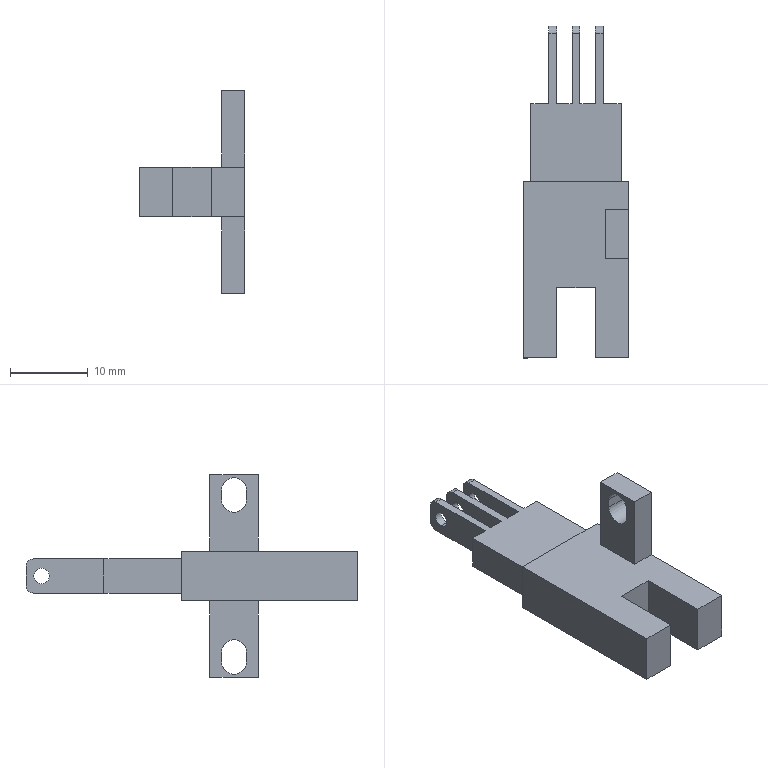Component | SolidWorks | U-shapedSensor8.28-1 | 1 solid | 55 faces | box 13.6 x 42.6 x 26 mm | volume 2610 mm3 | plane 39 | cylinder 16 | commonest cylinder face diameters 2 x12 3.2 x4
build123d program:
from build123d import *

# Parameters (mm, degrees)
SKETCH1_W              = 13.6
SKETCH1_H              = 22.6
BOSS_EXTRUDE1_DEPTH    = 6.4
SKETCH2_W              = 4.9
SKETCH2_H              = 9
CUT_EXTRUDE1_DEPTH     = 28.142
SKETCH3_W              = 13
SKETCH3_H              = 6.2
BOSS_EXTRUDE2_DEPTH    = 3
CUT_EXTRUDE2_DEPTH     = 31.954
SKETCH5_W              = 11.6
SKETCH5_H              = 4.4
BOSS_EXTRUDE3_DEPTH    = 10
SKETCH6_W              = 1
SKETCH6_H              = 4.4
BOSS_EXTRUDE4_DEPTH    = 10
FILLET1_R              = 1
SKETCH7_R              = 1
CUT_EXTRUDE3_DEPTH     = 10
LPATTERN1_COUNT        = 2
LPATTERN1_PITCH        = 3
LPATTERN1_COUNT_DIR2   = 2
LPATTERN1_PITCH_DIR2   = 3
FILLET1_OF_LPATTERN1_R = 1


with BuildPart() as part:
    # Sketch1 → Boss-Extrude1 (new body)
    with BuildSketch(Plane.XY):
        with Locations((6.8, -11.3)):
            Rectangle(SKETCH1_W, SKETCH1_H)
    extrude(amount=BOSS_EXTRUDE1_DEPTH)

    # Sketch2 → Cut-Extrude1 (cut, through all)
    with BuildSketch(Plane.XY.offset(6.4)):
        with Locations((6.8, -4.5)):
            Rectangle(SKETCH2_W, SKETCH2_H)
    extrude(amount=-CUT_EXTRUDE1_DEPTH, mode=Mode.SUBTRACT)

    # Sketch3 → Boss-Extrude2 (add)
    with BuildSketch(Plane.ZY):
        with Locations((9.7, -15.9)):
            Rectangle(SKETCH3_W, SKETCH3_H)
    boss_extrude2 = extrude(amount=-BOSS_EXTRUDE2_DEPTH)

    # Sketch4 → Cut-Extrude2 (cut, through all)
    with BuildSketch(Plane.ZY):
        with BuildLine():
            Line((13, -14.3), (14.2, -14.3))
            ThreePointArc((14.2, -14.3), (15.8, -15.9), (14.2, -17.5))
            Line((14.2, -17.5), (13, -17.5))
            ThreePointArc((13, -17.5), (11.4, -15.9), (13, -14.3))
        make_face()
    cut_extrude2 = extrude(amount=-CUT_EXTRUDE2_DEPTH, mode=Mode.SUBTRACT)

    # Mirror1: Boss-Extrude2, Cut-Extrude2 across plane
    add(boss_extrude2.mirror(Plane(origin=(0, 0, 3.2), x_dir=(1, 0, 0), z_dir=(0, 0, -1))))
    add(cut_extrude2.mirror(Plane(origin=(0, 0, 3.2), x_dir=(1, 0, 0), z_dir=(0, 0, -1))), mode=Mode.SUBTRACT)

    # Sketch5 → Boss-Extrude3 (add)
    with BuildSketch(Plane.XZ.offset(22.6)):
        with Locations((6.8, 3.2)):
            Rectangle(SKETCH5_W, SKETCH5_H)
    extrude(amount=BOSS_EXTRUDE3_DEPTH)

    # Sketch6 → Boss-Extrude4 (add)
    with BuildSketch(Plane.XZ.offset(32.6)):
        with Locations((6.8, 3.2)):
            Rectangle(SKETCH6_W, SKETCH6_H)
    boss_extrude4 = extrude(amount=BOSS_EXTRUDE4_DEPTH)

    # Fillet1
    fillet1_edges = [part.edges().sort_by_distance(p)[0] for p in [
        (6.8, -42.6, 1),
        (6.8, -42.6, 5.4),
    ]]
    fillet(fillet1_edges, radius=FILLET1_R)

    # Sketch7 → Cut-Extrude3 (cut)
    with BuildSketch(Plane.ZY.offset(-6.3)):
        with Locations((3.2, -40.6)):
            Circle(SKETCH7_R)
    cut_extrude3 = extrude(amount=-CUT_EXTRUDE3_DEPTH, mode=Mode.SUBTRACT)

    # LPattern1: Boss-Extrude4, Cut-Extrude3 2 × 2
    with Locations(*[Vector(1, 0, 0) * (i * LPATTERN1_PITCH) + Vector(-1, 0, 0) * (j * LPATTERN1_PITCH_DIR2) for i in range(LPATTERN1_COUNT) for j in range(LPATTERN1_COUNT_DIR2) if (i, j) != (0, 0)]):
        add(boss_extrude4)
        add(cut_extrude3, mode=Mode.SUBTRACT)

    # Fillet1 of LPattern1
    fillet1_of_lpattern1_edges = [part.edges().sort_by_distance(p)[0] for p in [
        (3.8, -42.6, 1),
        (3.8, -42.6, 5.4),
        (9.8, -42.6, 1),
        (9.8, -42.6, 5.4),
        (6.8, -42.6, 1),
        (6.8, -42.6, 5.4),
    ]]
    fillet(fillet1_of_lpattern1_edges, radius=FILLET1_OF_LPATTERN1_R)


solid = part.part

# Placed as in the assembly
solid = solid.moved(Location((-34.295, 69.645, -98.649), (0, 0, 180)))